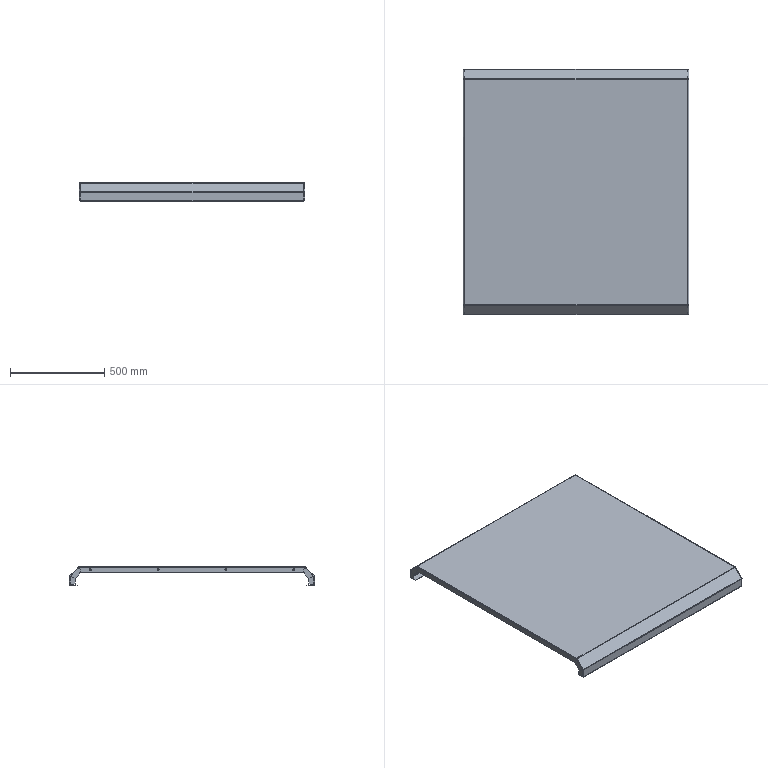Component | SolidWorks | MiddleTopCoverAssembly-1_MiddleTopCover-1 | 1 solid | 210 faces | volume 3754921 mm3 | plane 134 | cylinder 60 | spline 16 | commonest cylinder face diameters 10 x28 8 x16 4 x16 | material Plain Carbon Steel